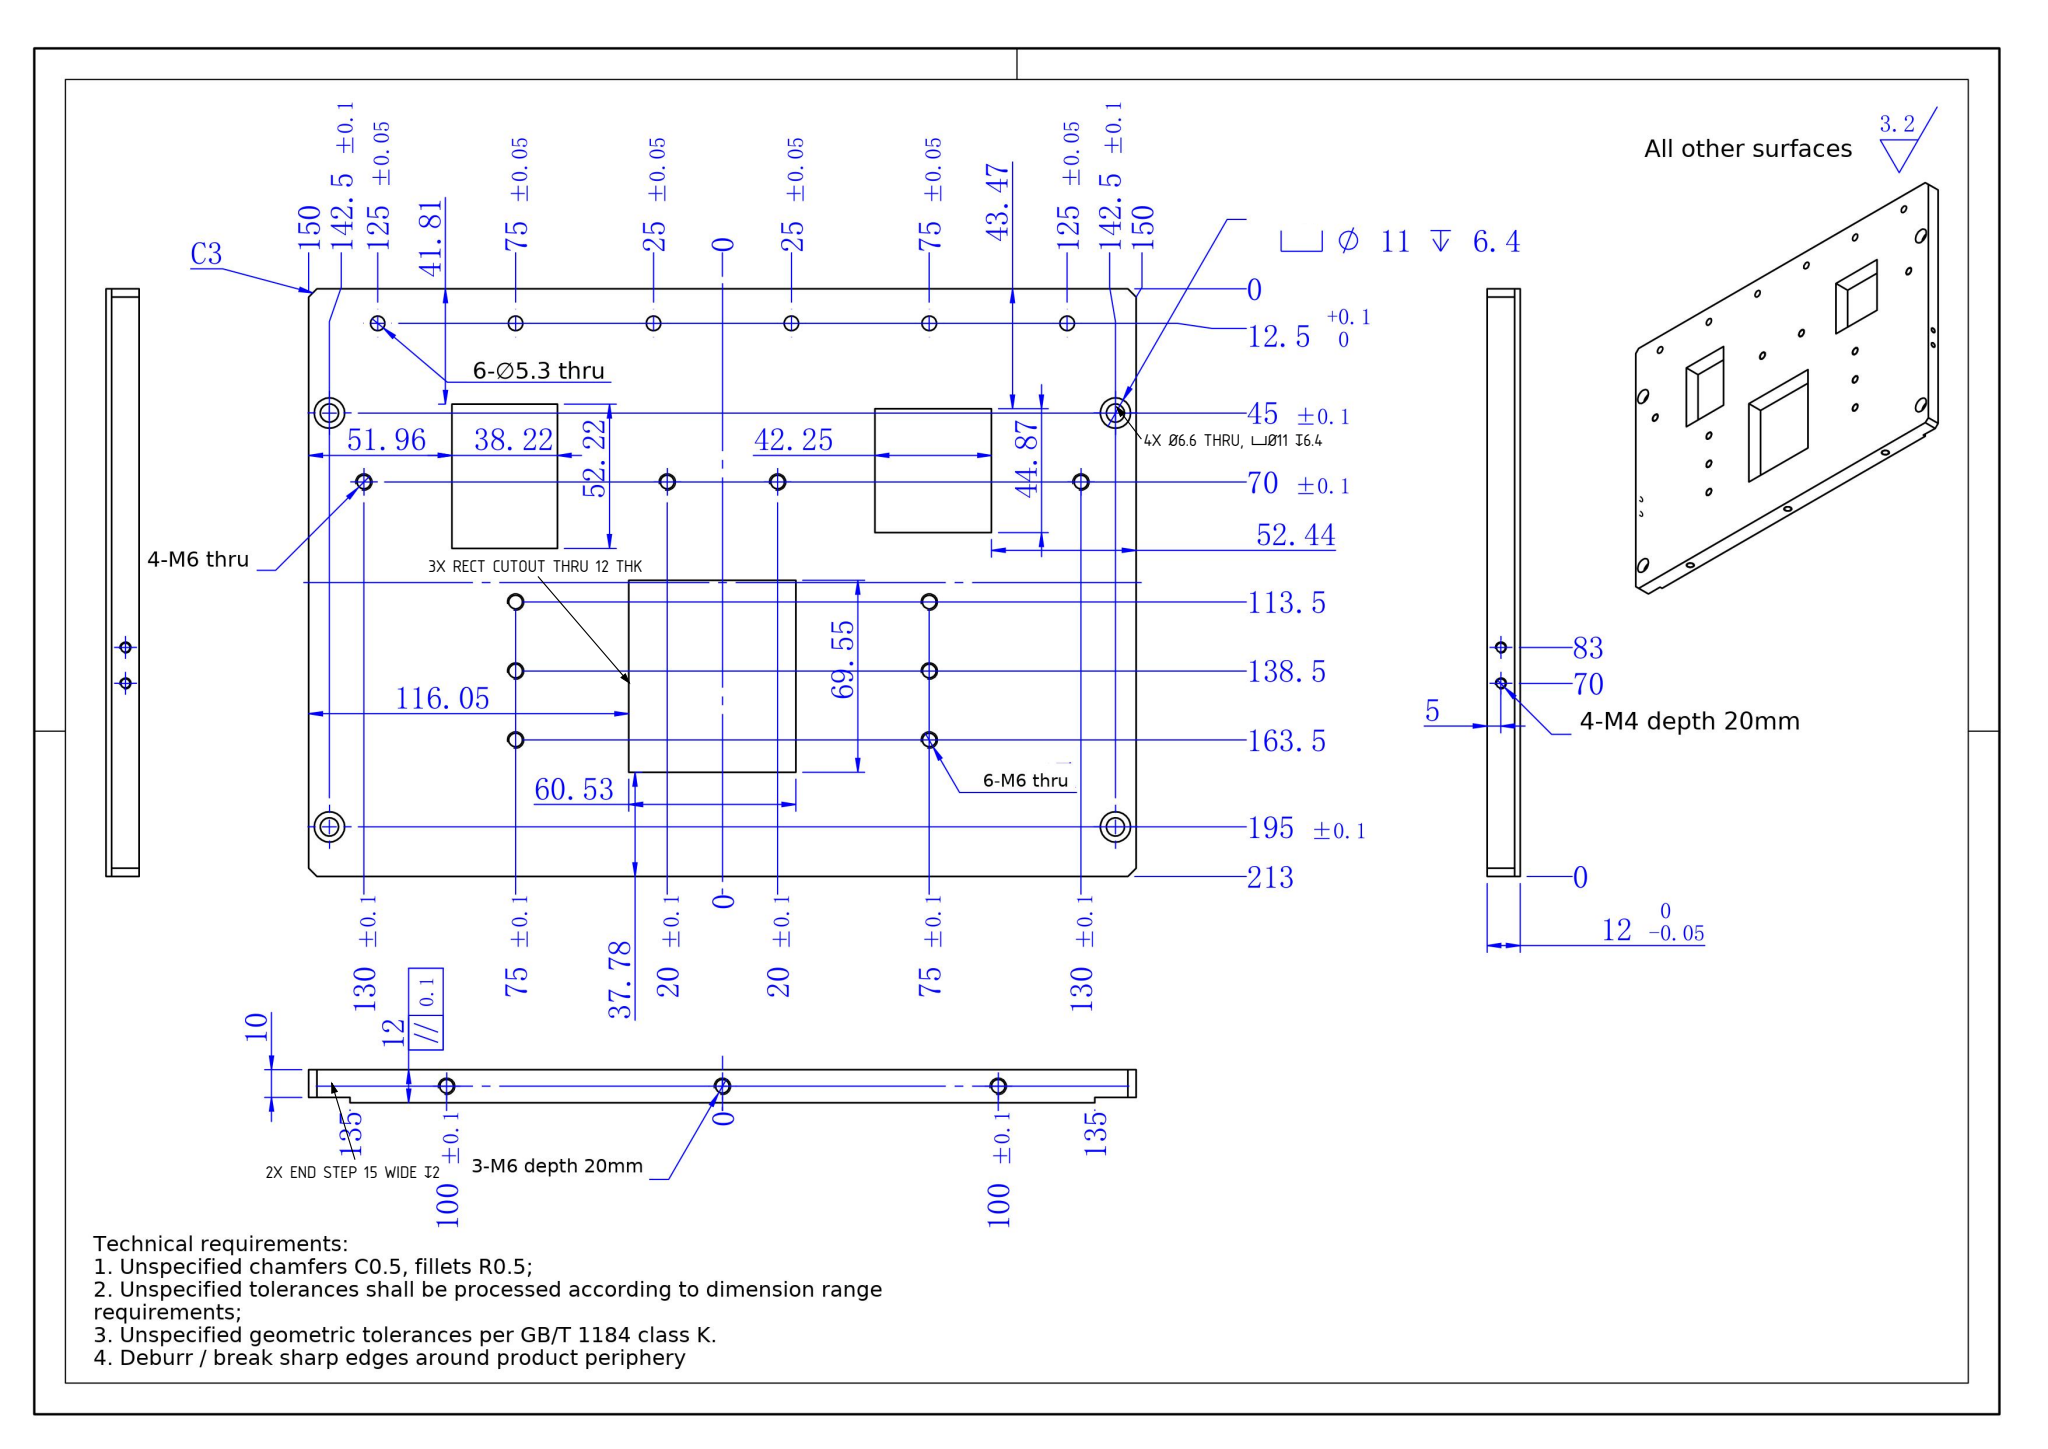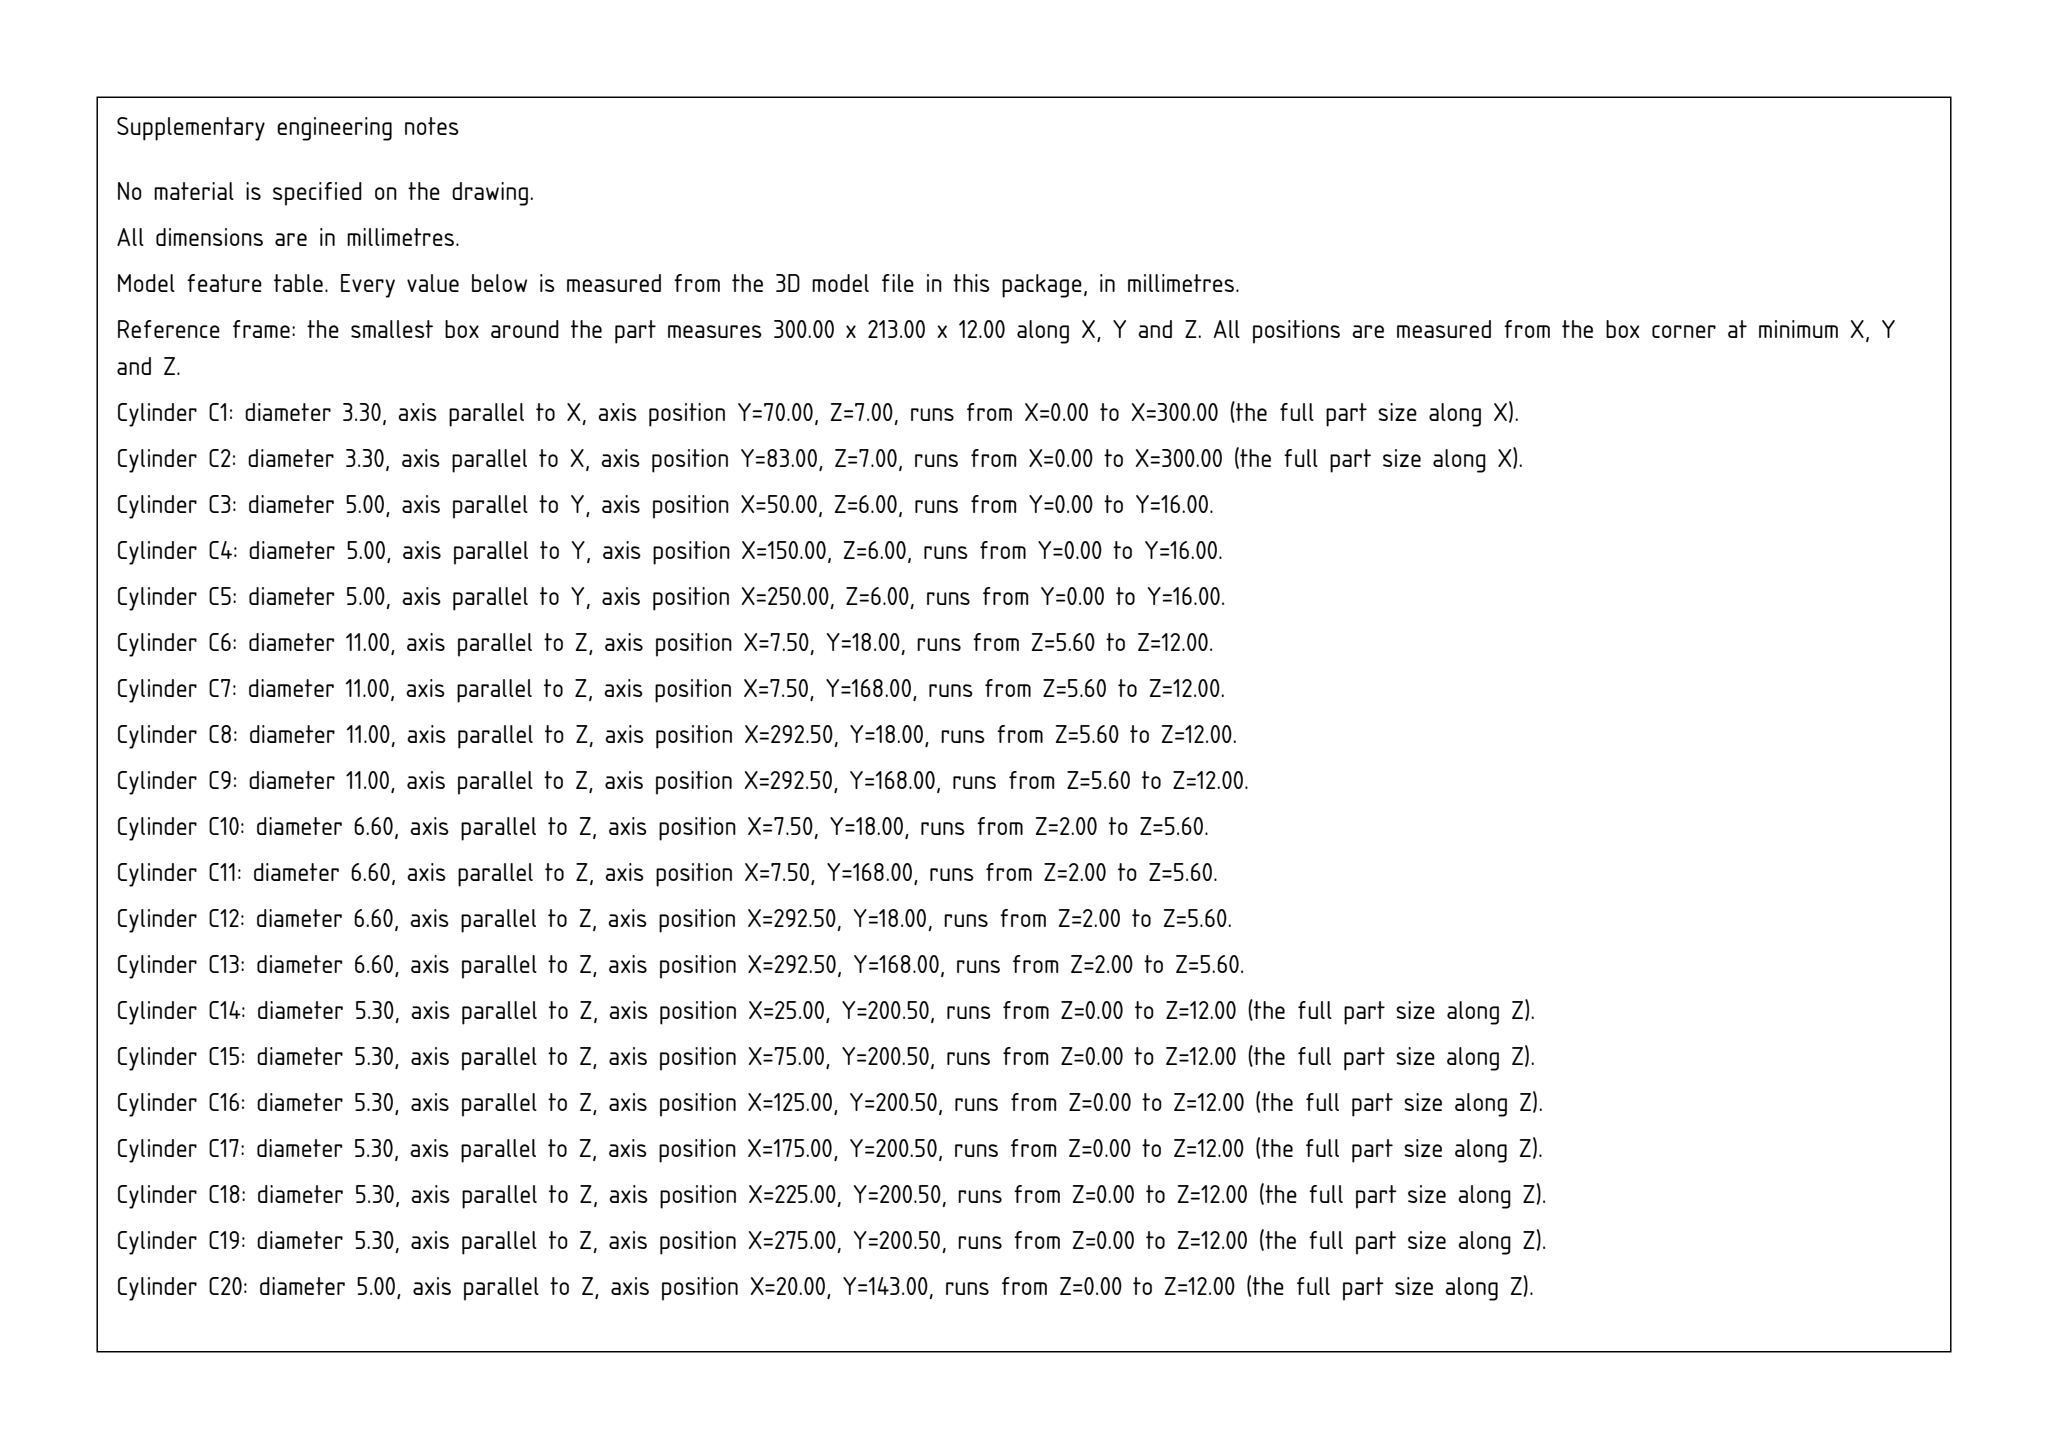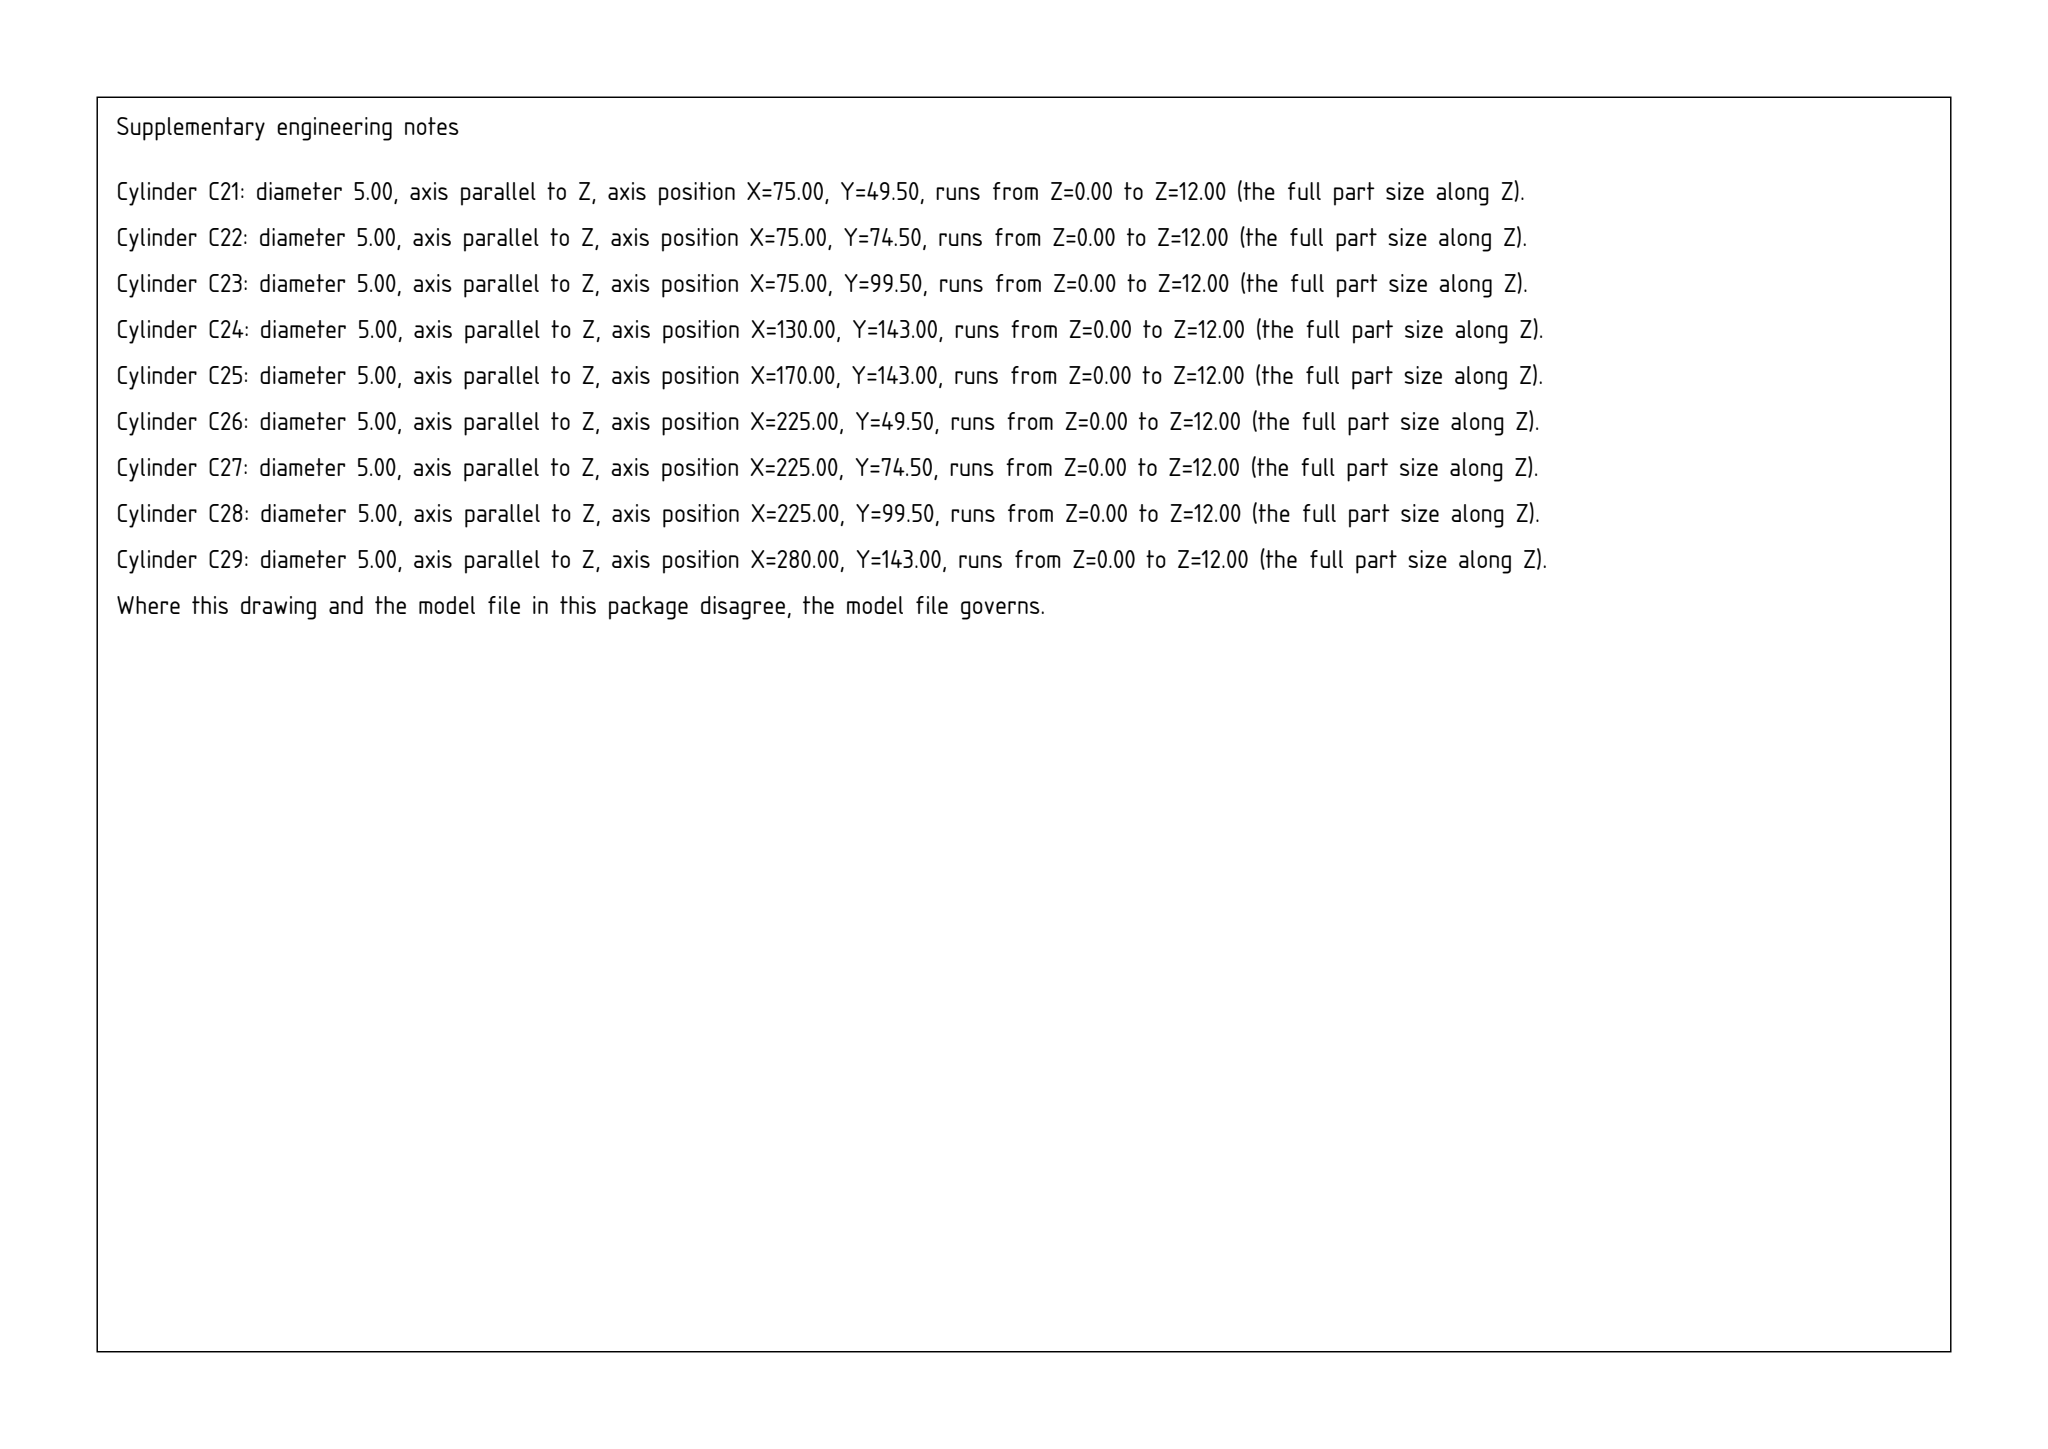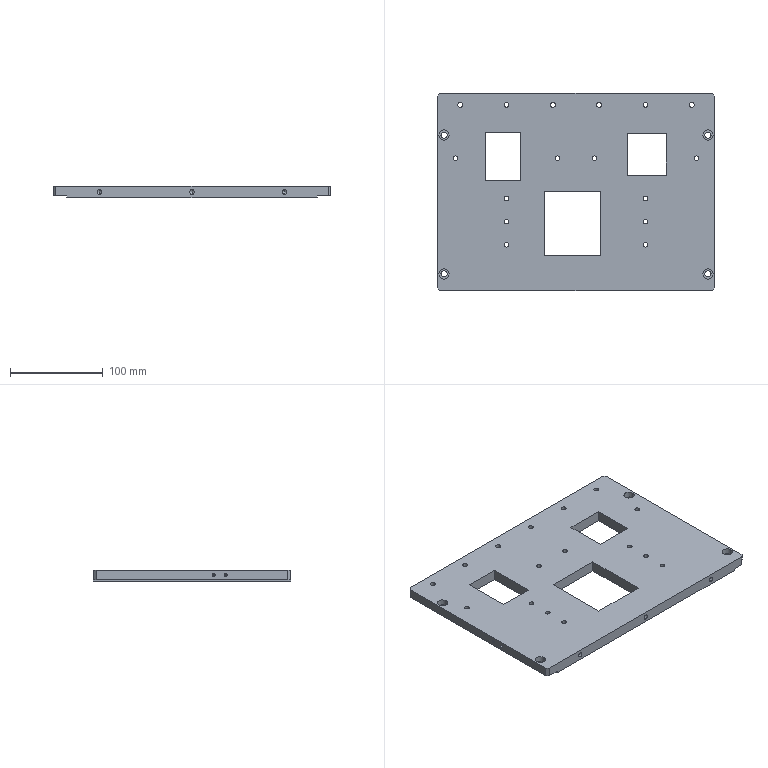Part | SolidWorks | mm | 1 solid | 106 faces | box 300 x 213 x 12 mm | volume 648080 mm3 | cylinder 62 | plane 30 | cone 14 | commonest cylinder face diameters 5 x26 5.3 x12 3.3 x8 11 x8 6.6 x8
Drawing notes:
END STEP: 15 WIDE x 2 DP EA END, 10 THK WALL REMAINING | from the solid: z planes 0/2/12 with x planes 0-15 & 285-300: 2 mm removed, 10 mm left
4X Ø6.6 THRU REMAINING 10 THK WALL, CBORE Ø11 DP 6.4 FROM TOP FACE; HOLES AT 7.5 AND 292.5 FROM LEFT EDGE, 18 AND 168 FROM BOTTOM EDGE (ALL FOUR CORNERS) | from the solid: cylinders: Ø6.6 z-axis at (7.5,18),(7.5,168),(292.5,18),(292.5,168) from z2.0 to 5.6; Ø11 same 4 positions from z5.6 to 12.0 (6.4 deep from z=12 top face)
ALL THREE RECTANGULAR CUTOUTS (38.22x52.22, 42.25x44.87, 60.53x69.55) ARE THRU, 12 THK PLATE | from the solid: axis_planes walls of pockets span z [0.0,12.0]: x52.0/x90.2 & y119.0/y171.2; x205.3/x247.6 & y124.7/y169.5; x116.1/x176.6 & y37.8/y107.3; plate bbox z=12.0
build123d program:
from build123d import *

# Parameters (mm, degrees)
SKETCH1_W                                       = 300
SKETCH1_H                                       = 213
EXTRUDE1_DEPTH                                  = 6
M6_TAPPED_HOLE1_D                               = 5
M6_TAPPED_HOLE1_DEPTH                           = 16
M6_TAPPED_HOLE1_TIP                             = 1.502
CHAMFER1_SIZE                                   = 3
M6_HEX_SOCKET_HEAD_CAP_SCREW_CBORE1_D           = 6.6
M6_HEX_SOCKET_HEAD_CAP_SCREW_CBORE1_CBORE_D     = 11
M6_HEX_SOCKET_HEAD_CAP_SCREW_CBORE1_CBORE_DEPTH = 6.4
SKETCH51_W                                      = 15
SKETCH51_H                                      = 2
CUT_EXTRUDE1_DEPTH                              = 318.222
F_5_3_5_3_DIAMETER_HOLE1_D                      = 5.3
M6_TAPPED_HOLE2_D                               = 5
M6_TAPPED_HOLE2_DEPTH                           = 15
M6_TAPPED_HOLE2_TIP                             = 1.502
M4_TAPPED_HOLE1_AT_2_COUNT                      = 2
M4_TAPPED_HOLE1_AT_2_PITCH                      = 13
M6_TAPPED_HOLE3_D                               = 5
M6_TAPPED_HOLE3_DEPTH                           = 15
M6_TAPPED_HOLE3_TIP                             = 1.502
SKETCH60_W                                      = 60.533
SKETCH60_H                                      = 69.553
SKETCH60_W_2                                    = 42.254
SKETCH60_H_2                                    = 44.865
SKETCH60_W_3                                    = 38.219
SKETCH60_H_3                                    = 52.224
CUT_EXTRUDE2_DEPTH                              = 125


with BuildPart() as part:
    # Sketch1 → Extrude1 (new, symmetric)
    with BuildSketch(Plane.XY):
        with Locations((85, -26.5)):
            Rectangle(SKETCH1_W, SKETCH1_H)
    extrude(amount=EXTRUDE1_DEPTH, both=True)

    # M6 Tapped Hole1
    with Locations(Plane.XZ.offset(133)):
        with Locations((-15, 0), (185, 0), (85, 0)):
            Hole(M6_TAPPED_HOLE1_D / 2, depth=M6_TAPPED_HOLE1_DEPTH)
            with Locations((0, 0, -(M6_TAPPED_HOLE1_DEPTH + M6_TAPPED_HOLE1_TIP / 2))):  # 118° drill point
                Cone(0, M6_TAPPED_HOLE1_D / 2, M6_TAPPED_HOLE1_TIP, mode=Mode.SUBTRACT)

    # Chamfer1
    chamfer1_edges = [part.edges().sort_by_distance(p)[0] for p in [
        (-65, 80, 0),
        (235, 80, 0),
        (235, -133, 0),
        (-65, -133, 0),
    ]]
    chamfer(chamfer1_edges, length=CHAMFER1_SIZE)

    # M6 Hex Socket Head Cap Screw CBORE1 (through all)
    with Locations(Plane.XY.offset(6)):
        with Locations((-57.5, 35), (-57.5, -115)):
            m6_hex_socket_head_cap_screw_cbore1 = CounterBoreHole(M6_HEX_SOCKET_HEAD_CAP_SCREW_CBORE1_D / 2, M6_HEX_SOCKET_HEAD_CAP_SCREW_CBORE1_CBORE_D / 2, M6_HEX_SOCKET_HEAD_CAP_SCREW_CBORE1_CBORE_DEPTH)

    # Mirror1: M6 Hex Socket Head Cap Screw CBORE1 across plane
    add(m6_hex_socket_head_cap_screw_cbore1.mirror(Plane(origin=(85, 0, 0), x_dir=(0, 0, 1), z_dir=(1, 0, 0))), mode=Mode.SUBTRACT)

    # Sketch51 → Cut-Extrude1 (cut, through all)
    with BuildSketch(Plane.XZ.offset(133)):
        with Locations((-57.5, -5)):
            Rectangle(SKETCH51_W, SKETCH51_H)
        with Locations((227.5, -5)):
            Rectangle(SKETCH51_W, SKETCH51_H)
    extrude(amount=-CUT_EXTRUDE1_DEPTH, mode=Mode.SUBTRACT)

    # 5.3 _5.3_ Diameter Hole1 (through all)
    with Locations(Plane(origin=(0, 0, -6), x_dir=(-1, 0, 0), z_dir=(0, 0, -1))):
        with Locations((-110, 67.5), (-160, 67.5), (-210, 67.5)):
            f_5_3_5_3_diameter_hole1 = Hole(F_5_3_5_3_DIAMETER_HOLE1_D / 2)

    # Mirror2: 5.3 _5.3_ Diameter Hole1 across plane
    add(f_5_3_5_3_diameter_hole1.mirror(Plane(origin=(85, 0, 0), x_dir=(0, 0, 1), z_dir=(1, 0, 0))), mode=Mode.SUBTRACT)

    # M6 Tapped Hole2
    with Locations(Plane.XY.offset(6)):
        with Locations((215, 10), (105, 10), (65, 10), (-45, 10)):
            Hole(M6_TAPPED_HOLE2_D / 2, depth=M6_TAPPED_HOLE2_DEPTH)
            with Locations((0, 0, -(M6_TAPPED_HOLE2_DEPTH + M6_TAPPED_HOLE2_TIP / 2))):  # 118° drill point
                Cone(0, M6_TAPPED_HOLE2_D / 2, M6_TAPPED_HOLE2_TIP, mode=Mode.SUBTRACT)

    # Sketch57 → M4 Tapped Hole1 (revolve, cut)
    with BuildSketch(Plane(origin=(235, -50, 1), x_dir=(0, 0, -1), z_dir=(0, 1, 0))):
        Polygon((0, 0), (0, 20.991), (1.65, 20), (1.65, 0), align=None)
    m4_tapped_hole1 = revolve(axis=Axis((241.35, -50, 1), (-1, 0, 0)), mode=Mode.SUBTRACT)

    # M4 Tapped Hole1 at 2: M4 Tapped Hole1 ×2
    with Locations(*[(0, -i * M4_TAPPED_HOLE1_AT_2_PITCH, 0) for i in range(1, M4_TAPPED_HOLE1_AT_2_COUNT)]):
        add(m4_tapped_hole1, mode=Mode.SUBTRACT)

    # Mirror3: M4 Tapped Hole1 across plane
    add(m4_tapped_hole1.mirror(Plane(origin=(85, 0, 0), x_dir=(0, 0, 1), z_dir=(1, 0, 0))), mode=Mode.SUBTRACT)

    # Mirror3 copy 1 sketch → Mirror3 copy 1 (revolve, cut)
    with BuildSketch(Plane(origin=(-65, -63, 1), x_dir=(0, 0, -1), z_dir=(0, 1, 0))):
        Polygon((0, 0), (0, -20.991), (1.65, -20), (1.65, 0), align=None)
    revolve(axis=Axis((-71.35, -63, 1), (-1, 0, 0)), mode=Mode.SUBTRACT)

    # M6 Tapped Hole3
    with Locations(Plane.XY.offset(6)):
        with Locations((10, -33.5), (10, -58.5), (10, -83.5), (160, -33.5), (160, -58.5), (160, -83.5)):
            Hole(M6_TAPPED_HOLE3_D / 2, depth=M6_TAPPED_HOLE3_DEPTH)
            with Locations((0, 0, -(M6_TAPPED_HOLE3_DEPTH + M6_TAPPED_HOLE3_TIP / 2))):  # 118° drill point
                Cone(0, M6_TAPPED_HOLE3_D / 2, M6_TAPPED_HOLE3_TIP, mode=Mode.SUBTRACT)

    # Sketch60 → Cut-Extrude2 (cut)
    with BuildSketch(Plane(origin=(0, 0, -6), x_dir=(-1, 0, 0), z_dir=(0, 0, -1))):
        with Locations((-81.321, -60.446)):
            Rectangle(SKETCH60_W, SKETCH60_H)
        with Locations((-161.437, 14.092)):
            Rectangle(SKETCH60_W_2, SKETCH60_H_2)
        with Locations((-6.07, 12.075)):
            Rectangle(SKETCH60_W_3, SKETCH60_H_3)
    extrude(amount=-CUT_EXTRUDE2_DEPTH, mode=Mode.SUBTRACT)


solid = part.part